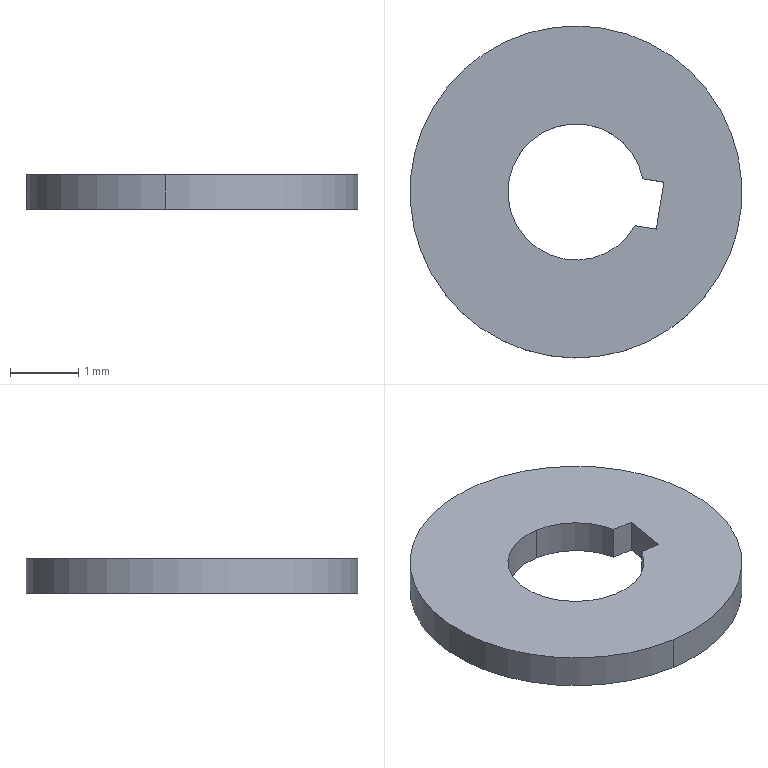Component | SolidWorks | Part29^Assembly1-2 | 1 solid | 10 faces | box 4.88 x 4.88 x 0.5 mm | volume 8 mm3 | cylinder 5 | plane 5 | commonest cylinder face diameters 2 x3 4.875 x2
STEP:
#1=COLOUR_RGB('',0.7922,0.8196,0.9333);
#2=FILL_AREA_STYLE_COLOUR('',#1);
#3=FILL_AREA_STYLE('',(#2));
#4=SURFACE_STYLE_FILL_AREA(#3);
#5=SURFACE_SIDE_STYLE('',(#4));
#6=SURFACE_STYLE_USAGE(.BOTH.,#5);
#7=PRESENTATION_STYLE_ASSIGNMENT((#6));
#8=CARTESIAN_POINT('',(0.4984,-0.09894,0.1969));
#9=VERTEX_POINT('',#8);
#10=CARTESIAN_POINT('',(0.4858,-0.1767,0.1969));
#11=VERTEX_POINT('',#10);
#12=CARTESIAN_POINT('',(0.4921,-0.1378,0.1969));
#13=DIRECTION('',(0.,-0.,1.));
#14=DIRECTION('',(-0.1605,-0.987,-0.));
#15=AXIS2_PLACEMENT_3D('',#12,#13,#14);
#16=CIRCLE('',#15,0.03937);
#17=EDGE_CURVE('',#9,#11,#16,.T.);
#18=ORIENTED_EDGE('',*,*,#17,.T.);
#19=CARTESIAN_POINT('',(0.4858,-0.1767,0.1772));
#20=VERTEX_POINT('',#19);
#21=CARTESIAN_POINT('',(0.4858,-0.1767,0.1969));
#22=DIRECTION('',(-0.,0.,-1.));
#23=VECTOR('',#22,39.37);
#24=LINE('',#21,#23);
#25=EDGE_CURVE('',#11,#20,#24,.T.);
#26=ORIENTED_EDGE('',*,*,#25,.T.);
#27=CARTESIAN_POINT('',(0.4984,-0.09894,0.1772));
#28=VERTEX_POINT('',#27);
#29=CARTESIAN_POINT('',(0.4921,-0.1378,0.1772));
#30=DIRECTION('',(0.,-0.,1.));
#31=DIRECTION('',(-0.1605,-0.987,-0.));
#32=AXIS2_PLACEMENT_3D('',#29,#30,#31);
#33=CIRCLE('',#32,0.03937);
#34=EDGE_CURVE('',#28,#20,#33,.T.);
#35=ORIENTED_EDGE('',*,*,#34,.F.);
#36=CARTESIAN_POINT('',(0.4984,-0.09894,0.1969));
#37=DIRECTION('',(-0.,0.,-1.));
#38=VECTOR('',#37,39.37);
#39=LINE('',#36,#38);
#40=EDGE_CURVE('',#9,#28,#39,.T.);
#41=ORIENTED_EDGE('',*,*,#40,.F.);
#42=EDGE_LOOP('',(#18,#26,#35,#41));
#43=FACE_OUTER_BOUND('',#42,.T.);
#44=CARTESIAN_POINT('',(0.4921,-0.1378,0.1969));
#45=DIRECTION('',(-0.,0.,-1.));
#46=DIRECTION('',(0.1605,0.987,0.));
#47=AXIS2_PLACEMENT_3D('',#44,#45,#46);
#48=CYLINDRICAL_SURFACE('',#47,0.03937);
#49=ADVANCED_FACE('',(#43),#48,.F.);
#50=CARTESIAN_POINT('',(0.5307,-0.1301,0.1969));
#51=VERTEX_POINT('',#50);
#52=CARTESIAN_POINT('',(0.4921,-0.1378,0.1969));
#53=DIRECTION('',(0.,-0.,1.));
#54=DIRECTION('',(-0.1605,-0.987,-0.));
#55=AXIS2_PLACEMENT_3D('',#52,#53,#54);
#56=CIRCLE('',#55,0.03937);
#57=EDGE_CURVE('',#51,#9,#56,.T.);
#58=ORIENTED_EDGE('',*,*,#57,.T.);
#59=ORIENTED_EDGE('',*,*,#40,.T.);
#60=CARTESIAN_POINT('',(0.5307,-0.1301,0.1772));
#61=VERTEX_POINT('',#60);
#62=CARTESIAN_POINT('',(0.4921,-0.1378,0.1772));
#63=DIRECTION('',(0.,-0.,1.));
#64=DIRECTION('',(-0.1605,-0.987,-0.));
#65=AXIS2_PLACEMENT_3D('',#62,#63,#64);
#66=CIRCLE('',#65,0.03937);
#67=EDGE_CURVE('',#61,#28,#66,.T.);
#68=ORIENTED_EDGE('',*,*,#67,.F.);
#69=CARTESIAN_POINT('',(0.5307,-0.1301,0.1969));
#70=DIRECTION('',(-0.,0.,-1.));
#71=VECTOR('',#70,39.37);
#72=LINE('',#69,#71);
#73=EDGE_CURVE('',#51,#61,#72,.T.);
#74=ORIENTED_EDGE('',*,*,#73,.F.);
#75=EDGE_LOOP('',(#58,#59,#68,#74));
#76=FACE_OUTER_BOUND('',#75,.T.);
#77=CARTESIAN_POINT('',(0.4921,-0.1378,0.1969));
#78=DIRECTION('',(-0.,0.,-1.));
#79=DIRECTION('',(0.1605,0.987,0.));
#80=AXIS2_PLACEMENT_3D('',#77,#78,#79);
#81=CYLINDRICAL_SURFACE('',#80,0.03937);
#82=ADVANCED_FACE('',(#76),#81,.F.);
#83=CARTESIAN_POINT('',(0.4767,-0.2325,0.1969));
#84=VERTEX_POINT('',#83);
#85=CARTESIAN_POINT('',(0.5075,-0.04307,0.1969));
#86=VERTEX_POINT('',#85);
#87=CARTESIAN_POINT('',(0.4921,-0.1378,0.1969));
#88=DIRECTION('',(0.,-0.,1.));
#89=DIRECTION('',(-0.1605,-0.987,-0.));
#90=AXIS2_PLACEMENT_3D('',#87,#88,#89);
#91=CIRCLE('',#90,0.09596);
#92=EDGE_CURVE('',#84,#86,#91,.T.);
#93=ORIENTED_EDGE('',*,*,#92,.F.);
#94=CARTESIAN_POINT('',(0.4767,-0.2325,0.1772));
#95=VERTEX_POINT('',#94);
#96=CARTESIAN_POINT('',(0.4767,-0.2325,0.1969));
#97=DIRECTION('',(-0.,0.,-1.));
#98=VECTOR('',#97,39.37);
#99=LINE('',#96,#98);
#100=EDGE_CURVE('',#84,#95,#99,.T.);
#101=ORIENTED_EDGE('',*,*,#100,.T.);
#102=CARTESIAN_POINT('',(0.5075,-0.04307,0.1772));
#103=VERTEX_POINT('',#102);
#104=CARTESIAN_POINT('',(0.4921,-0.1378,0.1772));
#105=DIRECTION('',(0.,-0.,1.));
#106=DIRECTION('',(-0.1605,-0.987,-0.));
#107=AXIS2_PLACEMENT_3D('',#104,#105,#106);
#108=CIRCLE('',#107,0.09596);
#109=EDGE_CURVE('',#95,#103,#108,.T.);
#110=ORIENTED_EDGE('',*,*,#109,.T.);
#111=CARTESIAN_POINT('',(0.5075,-0.04307,0.1969));
#112=DIRECTION('',(-0.,0.,-1.));
#113=VECTOR('',#112,39.37);
#114=LINE('',#111,#113);
#115=EDGE_CURVE('',#86,#103,#114,.T.);
#116=ORIENTED_EDGE('',*,*,#115,.F.);
#117=EDGE_LOOP('',(#93,#101,#110,#116));
#118=FACE_OUTER_BOUND('',#117,.T.);
#119=CARTESIAN_POINT('',(0.4921,-0.1378,0.1969));
#120=DIRECTION('',(-0.,0.,-1.));
#121=DIRECTION('',(0.1605,0.987,0.));
#122=AXIS2_PLACEMENT_3D('',#119,#120,#121);
#123=CYLINDRICAL_SURFACE('',#122,0.09596);
#124=ADVANCED_FACE('',(#118),#123,.T.);
#125=CARTESIAN_POINT('',(0.5263,-0.1573,0.1969));
#126=VERTEX_POINT('',#125);
#127=CARTESIAN_POINT('',(0.5385,-0.1593,0.1969));
#128=VERTEX_POINT('',#127);
#129=CARTESIAN_POINT('',(0.5385,-0.1593,0.1969));
#130=DIRECTION('',(0.987,-0.1605,-0.));
#131=VECTOR('',#130,39.37);
#132=LINE('',#129,#131);
#133=EDGE_CURVE('',#126,#128,#132,.T.);
#134=ORIENTED_EDGE('',*,*,#133,.F.);
#135=CARTESIAN_POINT('',(0.4921,-0.1378,0.1969));
#136=DIRECTION('',(0.,-0.,1.));
#137=DIRECTION('',(-0.1605,-0.987,-0.));
#138=AXIS2_PLACEMENT_3D('',#135,#136,#137);
#139=CIRCLE('',#138,0.03937);
#140=EDGE_CURVE('',#11,#126,#139,.T.);
#141=ORIENTED_EDGE('',*,*,#140,.F.);
#142=ORIENTED_EDGE('',*,*,#17,.F.);
#143=ORIENTED_EDGE('',*,*,#57,.F.);
#144=CARTESIAN_POINT('',(0.5429,-0.1321,0.1969));
#145=VERTEX_POINT('',#144);
#146=CARTESIAN_POINT('',(0.5429,-0.1321,0.1969));
#147=DIRECTION('',(-0.987,0.1605,0.));
#148=VECTOR('',#147,39.37);
#149=LINE('',#146,#148);
#150=EDGE_CURVE('',#145,#51,#149,.T.);
#151=ORIENTED_EDGE('',*,*,#150,.F.);
#152=CARTESIAN_POINT('',(0.5429,-0.1321,0.1969));
#153=DIRECTION('',(0.1605,0.987,0.));
#154=VECTOR('',#153,39.37);
#155=LINE('',#152,#154);
#156=EDGE_CURVE('',#128,#145,#155,.T.);
#157=ORIENTED_EDGE('',*,*,#156,.F.);
#158=EDGE_LOOP('',(#134,#141,#142,#143,#151,#157));
#159=FACE_BOUND('',#158,.T.);
#160=CARTESIAN_POINT('',(0.4921,-0.1378,0.1969));
#161=DIRECTION('',(0.,-0.,1.));
#162=DIRECTION('',(-0.1605,-0.987,-0.));
#163=AXIS2_PLACEMENT_3D('',#160,#161,#162);
#164=CIRCLE('',#163,0.09596);
#165=EDGE_CURVE('',#86,#84,#164,.T.);
#166=ORIENTED_EDGE('',*,*,#165,.T.);
#167=ORIENTED_EDGE('',*,*,#92,.T.);
#168=EDGE_LOOP('',(#166,#167));
#169=FACE_OUTER_BOUND('',#168,.T.);
#170=CARTESIAN_POINT('',(0.4921,-0.1378,0.1969));
#171=DIRECTION('',(0.,-0.,1.));
#172=DIRECTION('',(-0.1605,-0.987,-0.));
#173=AXIS2_PLACEMENT_3D('',#170,#171,#172);
#174=PLANE('',#173);
#175=ADVANCED_FACE('',(#159,#169),#174,.T.);
#176=ORIENTED_EDGE('',*,*,#67,.T.);
#177=ORIENTED_EDGE('',*,*,#34,.T.);
#178=CARTESIAN_POINT('',(0.5263,-0.1573,0.1772));
#179=VERTEX_POINT('',#178);
#180=CARTESIAN_POINT('',(0.4921,-0.1378,0.1772));
#181=DIRECTION('',(0.,-0.,1.));
#182=DIRECTION('',(-0.1605,-0.987,-0.));
#183=AXIS2_PLACEMENT_3D('',#180,#181,#182);
#184=CIRCLE('',#183,0.03937);
#185=EDGE_CURVE('',#20,#179,#184,.T.);
#186=ORIENTED_EDGE('',*,*,#185,.T.);
#187=CARTESIAN_POINT('',(0.5385,-0.1593,0.1772));
#188=VERTEX_POINT('',#187);
#189=CARTESIAN_POINT('',(0.4899,-0.1514,0.1772));
#190=DIRECTION('',(0.987,-0.1605,-0.));
#191=VECTOR('',#190,39.37);
#192=LINE('',#189,#191);
#193=EDGE_CURVE('',#179,#188,#192,.T.);
#194=ORIENTED_EDGE('',*,*,#193,.T.);
#195=CARTESIAN_POINT('',(0.5429,-0.1321,0.1772));
#196=VERTEX_POINT('',#195);
#197=CARTESIAN_POINT('',(0.5407,-0.1457,0.1772));
#198=DIRECTION('',(0.1605,0.987,0.));
#199=VECTOR('',#198,39.37);
#200=LINE('',#197,#199);
#201=EDGE_CURVE('',#188,#196,#200,.T.);
#202=ORIENTED_EDGE('',*,*,#201,.T.);
#203=CARTESIAN_POINT('',(0.4943,-0.1242,0.1772));
#204=DIRECTION('',(-0.987,0.1605,0.));
#205=VECTOR('',#204,39.37);
#206=LINE('',#203,#205);
#207=EDGE_CURVE('',#196,#61,#206,.T.);
#208=ORIENTED_EDGE('',*,*,#207,.T.);
#209=EDGE_LOOP('',(#176,#177,#186,#194,#202,#208));
#210=FACE_BOUND('',#209,.T.);
#211=CARTESIAN_POINT('',(0.4921,-0.1378,0.1772));
#212=DIRECTION('',(0.,-0.,1.));
#213=DIRECTION('',(-0.1605,-0.987,-0.));
#214=AXIS2_PLACEMENT_3D('',#211,#212,#213);
#215=CIRCLE('',#214,0.09596);
#216=EDGE_CURVE('',#103,#95,#215,.T.);
#217=ORIENTED_EDGE('',*,*,#216,.F.);
#218=ORIENTED_EDGE('',*,*,#109,.F.);
#219=EDGE_LOOP('',(#217,#218));
#220=FACE_OUTER_BOUND('',#219,.T.);
#221=CARTESIAN_POINT('',(0.4921,-0.1378,0.1772));
#222=DIRECTION('',(0.,-0.,1.));
#223=DIRECTION('',(-0.1605,-0.987,-0.));
#224=AXIS2_PLACEMENT_3D('',#221,#222,#223);
#225=PLANE('',#224);
#226=ADVANCED_FACE('',(#210,#220),#225,.F.);
#227=ORIENTED_EDGE('',*,*,#100,.F.);
#228=ORIENTED_EDGE('',*,*,#165,.F.);
#229=ORIENTED_EDGE('',*,*,#115,.T.);
#230=ORIENTED_EDGE('',*,*,#216,.T.);
#231=EDGE_LOOP('',(#227,#228,#229,#230));
#232=FACE_OUTER_BOUND('',#231,.T.);
#233=CARTESIAN_POINT('',(0.4921,-0.1378,0.1969));
#234=DIRECTION('',(-0.,0.,-1.));
#235=DIRECTION('',(0.1605,0.987,0.));
#236=AXIS2_PLACEMENT_3D('',#233,#234,#235);
#237=CYLINDRICAL_SURFACE('',#236,0.09596);
#238=ADVANCED_FACE('',(#232),#237,.T.);
#239=ORIENTED_EDGE('',*,*,#25,.F.);
#240=ORIENTED_EDGE('',*,*,#140,.T.);
#241=CARTESIAN_POINT('',(0.5263,-0.1573,0.1969));
#242=DIRECTION('',(0.,-0.,1.));
#243=VECTOR('',#242,39.37);
#244=LINE('',#241,#243);
#245=EDGE_CURVE('',#179,#126,#244,.T.);
#246=ORIENTED_EDGE('',*,*,#245,.F.);
#247=ORIENTED_EDGE('',*,*,#185,.F.);
#248=EDGE_LOOP('',(#239,#240,#246,#247));
#249=FACE_OUTER_BOUND('',#248,.T.);
#250=CARTESIAN_POINT('',(0.4921,-0.1378,0.1969));
#251=DIRECTION('',(-0.,0.,-1.));
#252=DIRECTION('',(0.1605,0.987,0.));
#253=AXIS2_PLACEMENT_3D('',#250,#251,#252);
#254=CYLINDRICAL_SURFACE('',#253,0.03937);
#255=ADVANCED_FACE('',(#249),#254,.F.);
#256=CARTESIAN_POINT('',(0.5385,-0.1593,0.1575));
#257=DIRECTION('',(0.,-0.,1.));
#258=VECTOR('',#257,39.37);
#259=LINE('',#256,#258);
#260=EDGE_CURVE('',#188,#128,#259,.T.);
#261=ORIENTED_EDGE('',*,*,#260,.T.);
#262=ORIENTED_EDGE('',*,*,#156,.T.);
#263=CARTESIAN_POINT('',(0.5429,-0.1321,0.1575));
#264=DIRECTION('',(0.,-0.,1.));
#265=VECTOR('',#264,39.37);
#266=LINE('',#263,#265);
#267=EDGE_CURVE('',#196,#145,#266,.T.);
#268=ORIENTED_EDGE('',*,*,#267,.F.);
#269=ORIENTED_EDGE('',*,*,#201,.F.);
#270=EDGE_LOOP('',(#261,#262,#268,#269));
#271=FACE_OUTER_BOUND('',#270,.T.);
#272=CARTESIAN_POINT('',(0.5429,-0.1321,0.1575));
#273=DIRECTION('',(0.987,-0.1605,-0.));
#274=DIRECTION('',(0.,-0.,1.));
#275=AXIS2_PLACEMENT_3D('',#272,#273,#274);
#276=PLANE('',#275);
#277=ADVANCED_FACE('',(#271),#276,.F.);
#278=ORIENTED_EDGE('',*,*,#245,.T.);
#279=ORIENTED_EDGE('',*,*,#133,.T.);
#280=ORIENTED_EDGE('',*,*,#260,.F.);
#281=ORIENTED_EDGE('',*,*,#193,.F.);
#282=EDGE_LOOP('',(#278,#279,#280,#281));
#283=FACE_OUTER_BOUND('',#282,.T.);
#284=CARTESIAN_POINT('',(0.5385,-0.1593,0.1575));
#285=DIRECTION('',(-0.1605,-0.987,-0.));
#286=DIRECTION('',(-0.,0.,-1.));
#287=AXIS2_PLACEMENT_3D('',#284,#285,#286);
#288=PLANE('',#287);
#289=ADVANCED_FACE('',(#283),#288,.F.);
#290=ORIENTED_EDGE('',*,*,#267,.T.);
#291=ORIENTED_EDGE('',*,*,#150,.T.);
#292=ORIENTED_EDGE('',*,*,#73,.T.);
#293=ORIENTED_EDGE('',*,*,#207,.F.);
#294=EDGE_LOOP('',(#290,#291,#292,#293));
#295=FACE_OUTER_BOUND('',#294,.T.);
#296=CARTESIAN_POINT('',(0.5429,-0.1321,0.1575));
#297=DIRECTION('',(0.1605,0.987,0.));
#298=DIRECTION('',(0.,-0.,1.));
#299=AXIS2_PLACEMENT_3D('',#296,#297,#298);
#300=PLANE('',#299);
#301=ADVANCED_FACE('',(#295),#300,.F.);
#302=CLOSED_SHELL('',(#49,#82,#124,#175,#226,#238,#255,#277,#289,#301));
#303=MANIFOLD_SOLID_BREP('',#302);
#304=STYLED_ITEM('',(#7),#303);
#305=PRESENTATION_LAYER_ASSIGNMENT('','',(#304));
#306=(LENGTH_UNIT()NAMED_UNIT(*)SI_UNIT($,.METRE.));
#307=LENGTH_MEASURE_WITH_UNIT(LENGTH_MEASURE(0.0254),#306);
#308=DIMENSIONAL_EXPONENTS(1.,0.,0.,0.,0.,0.,0.);
#309=(CONVERSION_BASED_UNIT('',#307)LENGTH_UNIT()NAMED_UNIT(#308));
#310=UNCERTAINTY_MEASURE_WITH_UNIT(LENGTH_MEASURE(0.00001),#309,'','');
#311=(NAMED_UNIT(*)PLANE_ANGLE_UNIT()SI_UNIT($,.RADIAN.));
#312=(NAMED_UNIT(*)SI_UNIT($,.STERADIAN.)SOLID_ANGLE_UNIT());
#313=(GEOMETRIC_REPRESENTATION_CONTEXT(3)GLOBAL_UNCERTAINTY_ASSIGNED_CONTEXT((#310))GLOBAL_UNIT_ASSIGNED_CONTEXT((#309,#311,#312))REPRESENTATION_CONTEXT('',''));
#314=MECHANICAL_DESIGN_GEOMETRIC_PRESENTATION_REPRESENTATION('',(#304),#313);
#315=CARTESIAN_POINT('',(0.,0.,0.));
#316=DIRECTION('',(0.,0.,1.));
#317=DIRECTION('',(1.,0.,0.));
#318=AXIS2_PLACEMENT_3D('',#315,#316,#317);
#319=(LENGTH_UNIT()NAMED_UNIT(*)SI_UNIT($,.METRE.));
#320=LENGTH_MEASURE_WITH_UNIT(LENGTH_MEASURE(0.0254),#319);
#321=DIMENSIONAL_EXPONENTS(1.,0.,0.,0.,0.,0.,0.);
#322=(CONVERSION_BASED_UNIT('',#320)LENGTH_UNIT()NAMED_UNIT(#321));
#323=UNCERTAINTY_MEASURE_WITH_UNIT(LENGTH_MEASURE(0.00001),#322,'','');
#324=(NAMED_UNIT(*)PLANE_ANGLE_UNIT()SI_UNIT($,.RADIAN.));
#325=(NAMED_UNIT(*)SI_UNIT($,.STERADIAN.)SOLID_ANGLE_UNIT());
#326=(GEOMETRIC_REPRESENTATION_CONTEXT(3)GLOBAL_UNCERTAINTY_ASSIGNED_CONTEXT((#323))GLOBAL_UNIT_ASSIGNED_CONTEXT((#322,#324,#325))REPRESENTATION_CONTEXT('',''));
#327=ADVANCED_BREP_SHAPE_REPRESENTATION('',(#303,#318),#326);